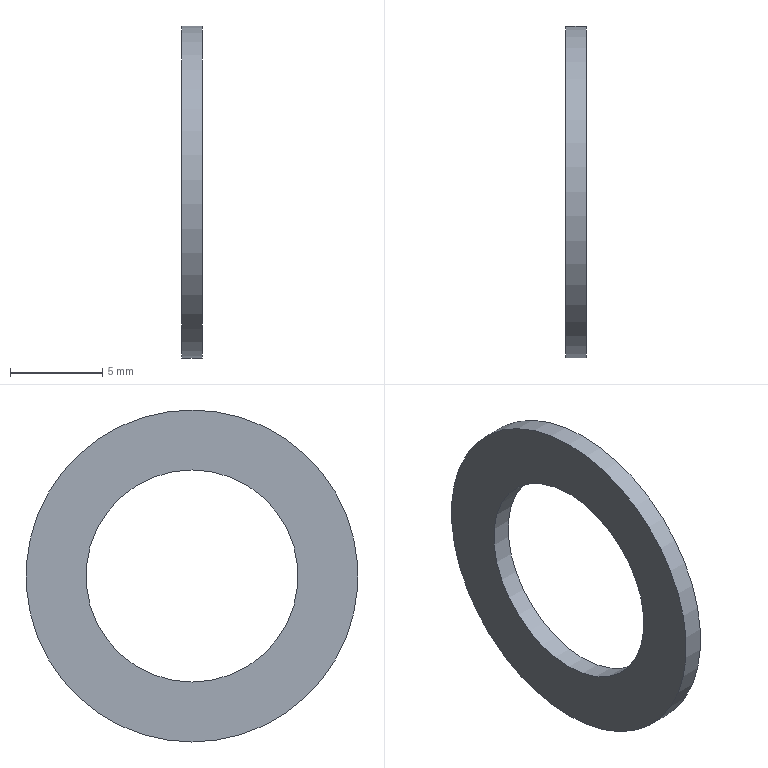Component | NX | RETAINING_RING | 1 solid | 4 faces | box 1.1 x 18 x 18 mm | volume 166 mm3 | cylinder 2 | plane 2 | commonest cylinder face diameters 18 x1 11.5 x1
STEP:
#1=CARTESIAN_POINT('',(0.,0.,0.));
#2=DIRECTION('',(0.,0.,1.));
#3=DIRECTION('',(1.,0.,0.));
#4=AXIS2_PLACEMENT_3D('',#1,#2,#3);
#5=CARTESIAN_POINT('',(22.4,0.,27.));
#6=VERTEX_POINT('',#5);
#7=CARTESIAN_POINT('',(22.4,0.,18.));
#8=DIRECTION('',(1.,0.,0.));
#9=DIRECTION('',(0.,0.,1.));
#10=AXIS2_PLACEMENT_3D('',#7,#8,#9);
#11=CIRCLE('',#10,9.);
#12=CARTESIAN_POINT('',(22.4,0.,18.));
#13=DIRECTION('',(1.,0.,0.));
#14=DIRECTION('',(0.,0.,-1.));
#15=AXIS2_PLACEMENT_3D('',#12,#13,#14);
#16=CYLINDRICAL_SURFACE('',#15,9.);
#17=CARTESIAN_POINT('',(3.142,0.));
#18=DIRECTION('',(1.,0.));
#19=VECTOR('',#18,1.);
#20=LINE('',#17,#19);
#21=(GEOMETRIC_REPRESENTATION_CONTEXT(2)PARAMETRIC_REPRESENTATION_CONTEXT()REPRESENTATION_CONTEXT('',''));
#22=DEFINITIONAL_REPRESENTATION('',(#20),#21);
#23=PCURVE('',#16,#22);
#24=CARTESIAN_POINT('',(22.4,0.,18.));
#25=DIRECTION('',(1.,0.,0.));
#26=DIRECTION('',(0.,0.,-1.));
#27=AXIS2_PLACEMENT_3D('',#24,#25,#26);
#28=PLANE('',#27);
#29=CARTESIAN_POINT('',(0.,0.));
#30=DIRECTION('',(-1.,0.));
#31=AXIS2_PLACEMENT_2D('',#29,#30);
#32=CIRCLE('',#31,9.);
#33=(GEOMETRIC_REPRESENTATION_CONTEXT(2)PARAMETRIC_REPRESENTATION_CONTEXT()REPRESENTATION_CONTEXT('',''));
#34=DEFINITIONAL_REPRESENTATION('',(#32),#33);
#35=PCURVE('',#28,#34);
#36=SURFACE_CURVE('',#11,(#23,#35),.PCURVE_S1.);
#37=EDGE_CURVE('',#6,#6,#36,.T.);
#38=ORIENTED_EDGE('',*,*,#37,.T.);
#39=CARTESIAN_POINT('',(23.5,0.,27.));
#40=VERTEX_POINT('',#39);
#41=CARTESIAN_POINT('',(22.4,0.,27.));
#42=CARTESIAN_POINT('',(23.5,0.,27.));
#43=B_SPLINE_CURVE_WITH_KNOTS('',1,(#41,#42),.UNSPECIFIED.,.F.,.F.,(2,2),(0.,1.1),.PIECEWISE_BEZIER_KNOTS.);
#44=CARTESIAN_POINT('',(9.425,0.));
#45=DIRECTION('',(0.,1.));
#46=VECTOR('',#45,1.);
#47=LINE('',#44,#46);
#48=(GEOMETRIC_REPRESENTATION_CONTEXT(2)PARAMETRIC_REPRESENTATION_CONTEXT()REPRESENTATION_CONTEXT('',''));
#49=DEFINITIONAL_REPRESENTATION('',(#47),#48);
#50=PCURVE('',#16,#49);
#51=CARTESIAN_POINT('',(3.142,0.));
#52=DIRECTION('',(0.,1.));
#53=VECTOR('',#52,1.);
#54=LINE('',#51,#53);
#55=(GEOMETRIC_REPRESENTATION_CONTEXT(2)PARAMETRIC_REPRESENTATION_CONTEXT()REPRESENTATION_CONTEXT('',''));
#56=DEFINITIONAL_REPRESENTATION('',(#54),#55);
#57=PCURVE('',#16,#56);
#58=SEAM_CURVE('',#43,(#50,#57),.PCURVE_S1.);
#59=EDGE_CURVE('',#6,#40,#58,.T.);
#60=ORIENTED_EDGE('',*,*,#59,.T.);
#61=CARTESIAN_POINT('',(23.5,0.,18.));
#62=DIRECTION('',(1.,0.,0.));
#63=DIRECTION('',(0.,0.,1.));
#64=AXIS2_PLACEMENT_3D('',#61,#62,#63);
#65=CIRCLE('',#64,9.);
#66=CARTESIAN_POINT('',(3.142,1.1));
#67=DIRECTION('',(1.,0.));
#68=VECTOR('',#67,1.);
#69=LINE('',#66,#68);
#70=(GEOMETRIC_REPRESENTATION_CONTEXT(2)PARAMETRIC_REPRESENTATION_CONTEXT()REPRESENTATION_CONTEXT('',''));
#71=DEFINITIONAL_REPRESENTATION('',(#69),#70);
#72=PCURVE('',#16,#71);
#73=CARTESIAN_POINT('',(23.5,0.,18.));
#74=DIRECTION('',(1.,0.,0.));
#75=DIRECTION('',(0.,0.,-1.));
#76=AXIS2_PLACEMENT_3D('',#73,#74,#75);
#77=PLANE('',#76);
#78=CARTESIAN_POINT('',(0.,0.));
#79=DIRECTION('',(-1.,0.));
#80=AXIS2_PLACEMENT_2D('',#78,#79);
#81=CIRCLE('',#80,9.);
#82=(GEOMETRIC_REPRESENTATION_CONTEXT(2)PARAMETRIC_REPRESENTATION_CONTEXT()REPRESENTATION_CONTEXT('',''));
#83=DEFINITIONAL_REPRESENTATION('',(#81),#82);
#84=PCURVE('',#77,#83);
#85=SURFACE_CURVE('',#65,(#72,#84),.PCURVE_S1.);
#86=EDGE_CURVE('',#40,#40,#85,.T.);
#87=ORIENTED_EDGE('',*,*,#86,.F.);
#88=ORIENTED_EDGE('',*,*,#59,.F.);
#89=EDGE_LOOP('',(#38,#60,#87,#88));
#90=FACE_BOUND('',#89,.T.);
#91=ADVANCED_FACE('',(#90),#16,.T.);
#92=CARTESIAN_POINT('',(22.4,0.,23.75));
#93=VERTEX_POINT('',#92);
#94=CARTESIAN_POINT('',(22.4,0.,18.));
#95=DIRECTION('',(1.,0.,0.));
#96=DIRECTION('',(0.,0.,1.));
#97=AXIS2_PLACEMENT_3D('',#94,#95,#96);
#98=CIRCLE('',#97,5.75);
#99=CARTESIAN_POINT('',(22.4,0.,18.));
#100=DIRECTION('',(1.,0.,0.));
#101=DIRECTION('',(0.,0.,-1.));
#102=AXIS2_PLACEMENT_3D('',#99,#100,#101);
#103=CYLINDRICAL_SURFACE('',#102,5.75);
#104=CARTESIAN_POINT('',(3.142,0.));
#105=DIRECTION('',(1.,0.));
#106=VECTOR('',#105,1.);
#107=LINE('',#104,#106);
#108=(GEOMETRIC_REPRESENTATION_CONTEXT(2)PARAMETRIC_REPRESENTATION_CONTEXT()REPRESENTATION_CONTEXT('',''));
#109=DEFINITIONAL_REPRESENTATION('',(#107),#108);
#110=PCURVE('',#103,#109);
#111=CARTESIAN_POINT('',(0.,0.));
#112=DIRECTION('',(-1.,0.));
#113=AXIS2_PLACEMENT_2D('',#111,#112);
#114=CIRCLE('',#113,5.75);
#115=(GEOMETRIC_REPRESENTATION_CONTEXT(2)PARAMETRIC_REPRESENTATION_CONTEXT()REPRESENTATION_CONTEXT('',''));
#116=DEFINITIONAL_REPRESENTATION('',(#114),#115);
#117=PCURVE('',#28,#116);
#118=SURFACE_CURVE('',#98,(#110,#117),.PCURVE_S1.);
#119=EDGE_CURVE('',#93,#93,#118,.T.);
#120=ORIENTED_EDGE('',*,*,#119,.T.);
#121=CARTESIAN_POINT('',(23.5,0.,23.75));
#122=VERTEX_POINT('',#121);
#123=CARTESIAN_POINT('',(22.4,0.,23.75));
#124=CARTESIAN_POINT('',(23.5,0.,23.75));
#125=B_SPLINE_CURVE_WITH_KNOTS('',1,(#123,#124),.UNSPECIFIED.,.F.,.F.,(2,2),(0.,1.1),.PIECEWISE_BEZIER_KNOTS.);
#126=CARTESIAN_POINT('',(9.425,0.));
#127=DIRECTION('',(0.,1.));
#128=VECTOR('',#127,1.);
#129=LINE('',#126,#128);
#130=(GEOMETRIC_REPRESENTATION_CONTEXT(2)PARAMETRIC_REPRESENTATION_CONTEXT()REPRESENTATION_CONTEXT('',''));
#131=DEFINITIONAL_REPRESENTATION('',(#129),#130);
#132=PCURVE('',#103,#131);
#133=CARTESIAN_POINT('',(3.142,0.));
#134=DIRECTION('',(0.,1.));
#135=VECTOR('',#134,1.);
#136=LINE('',#133,#135);
#137=(GEOMETRIC_REPRESENTATION_CONTEXT(2)PARAMETRIC_REPRESENTATION_CONTEXT()REPRESENTATION_CONTEXT('',''));
#138=DEFINITIONAL_REPRESENTATION('',(#136),#137);
#139=PCURVE('',#103,#138);
#140=SEAM_CURVE('',#125,(#132,#139),.PCURVE_S1.);
#141=EDGE_CURVE('',#93,#122,#140,.T.);
#142=ORIENTED_EDGE('',*,*,#141,.T.);
#143=CARTESIAN_POINT('',(23.5,0.,18.));
#144=DIRECTION('',(1.,0.,0.));
#145=DIRECTION('',(0.,0.,1.));
#146=AXIS2_PLACEMENT_3D('',#143,#144,#145);
#147=CIRCLE('',#146,5.75);
#148=CARTESIAN_POINT('',(3.142,1.1));
#149=DIRECTION('',(1.,0.));
#150=VECTOR('',#149,1.);
#151=LINE('',#148,#150);
#152=(GEOMETRIC_REPRESENTATION_CONTEXT(2)PARAMETRIC_REPRESENTATION_CONTEXT()REPRESENTATION_CONTEXT('',''));
#153=DEFINITIONAL_REPRESENTATION('',(#151),#152);
#154=PCURVE('',#103,#153);
#155=CARTESIAN_POINT('',(0.,0.));
#156=DIRECTION('',(-1.,0.));
#157=AXIS2_PLACEMENT_2D('',#155,#156);
#158=CIRCLE('',#157,5.75);
#159=(GEOMETRIC_REPRESENTATION_CONTEXT(2)PARAMETRIC_REPRESENTATION_CONTEXT()REPRESENTATION_CONTEXT('',''));
#160=DEFINITIONAL_REPRESENTATION('',(#158),#159);
#161=PCURVE('',#77,#160);
#162=SURFACE_CURVE('',#147,(#154,#161),.PCURVE_S1.);
#163=EDGE_CURVE('',#122,#122,#162,.T.);
#164=ORIENTED_EDGE('',*,*,#163,.F.);
#165=ORIENTED_EDGE('',*,*,#141,.F.);
#166=EDGE_LOOP('',(#120,#142,#164,#165));
#167=FACE_BOUND('',#166,.F.);
#168=ADVANCED_FACE('',(#167),#103,.F.);
#169=ORIENTED_EDGE('',*,*,#37,.F.);
#170=EDGE_LOOP('',(#169));
#171=FACE_BOUND('',#170,.T.);
#172=ORIENTED_EDGE('',*,*,#119,.T.);
#173=EDGE_LOOP('',(#172));
#174=FACE_BOUND('',#173,.T.);
#175=ADVANCED_FACE('',(#171,#174),#28,.F.);
#176=ORIENTED_EDGE('',*,*,#86,.T.);
#177=EDGE_LOOP('',(#176));
#178=FACE_BOUND('',#177,.T.);
#179=ORIENTED_EDGE('',*,*,#163,.F.);
#180=EDGE_LOOP('',(#179));
#181=FACE_BOUND('',#180,.T.);
#182=ADVANCED_FACE('',(#178,#181),#77,.T.);
#183=CLOSED_SHELL('',(#91,#168,#175,#182));
#184=MANIFOLD_SOLID_BREP('',#183);
#185=(LENGTH_UNIT()NAMED_UNIT(*)SI_UNIT(.MILLI.,.METRE.));
#186=UNCERTAINTY_MEASURE_WITH_UNIT(LENGTH_MEASURE(0.00001),#185,'','');
#187=(NAMED_UNIT(*)PLANE_ANGLE_UNIT()SI_UNIT($,.RADIAN.));
#188=(NAMED_UNIT(*)SI_UNIT($,.STERADIAN.)SOLID_ANGLE_UNIT());
#189=(GEOMETRIC_REPRESENTATION_CONTEXT(3)GLOBAL_UNCERTAINTY_ASSIGNED_CONTEXT((#186))GLOBAL_UNIT_ASSIGNED_CONTEXT((#185,#187,#188))REPRESENTATION_CONTEXT('',''));
#190=ADVANCED_BREP_SHAPE_REPRESENTATION('',(#4,#184),#189);